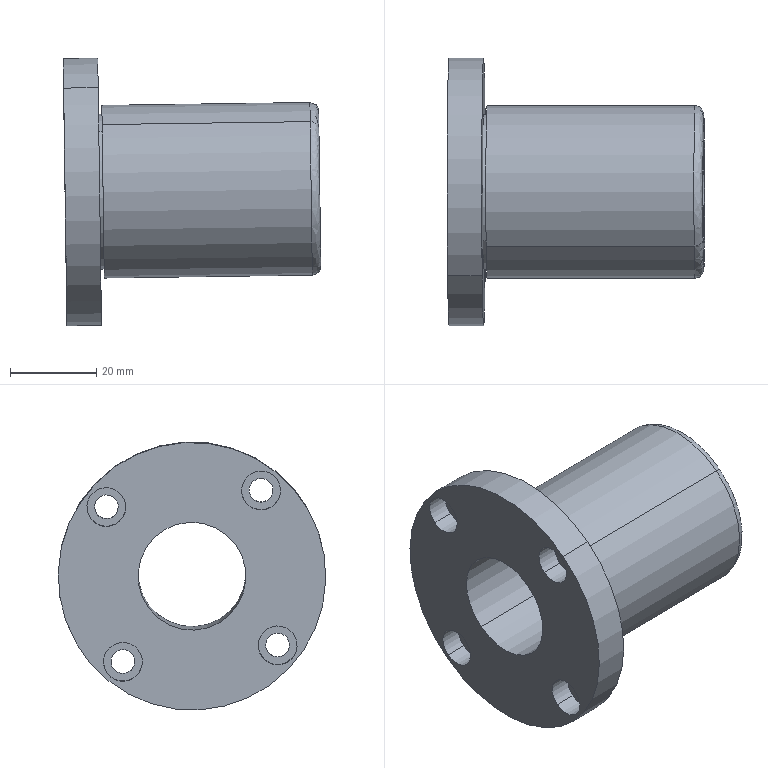Component | SolidWorks | DA-0220-LHFR25-18 | 1 solid | 34 faces | box 59.68 x 62 x 62.11 mm | volume 57411 mm3 | cylinder 24 | plane 8 | spline 2 | commonest cylinder face diameters 5.5 x8 9 x8 40 x2 36 x2 25 x2 62 x2
STEP:
#1=CARTESIAN_POINT('',(34.201,-7.018,18.749));
#2=VERTEX_POINT('',#1);
#3=CARTESIAN_POINT('',(34.218,-6.029,17.524));
#4=VERTEX_POINT('',#3);
#5=CARTESIAN_POINT('',(34.209,-6.524,18.137));
#6=DIRECTION('',(-0.9999,-0.000404,-0.01395));
#7=DIRECTION('',(-0.01061,-0.628,0.7781));
#8=AXIS2_PLACEMENT_3D('',#5,#6,#7);
#9=CIRCLE('',#8,0.7874);
#10=EDGE_CURVE('',#2,#4,#9,.T.);
#11=ORIENTED_EDGE('',*,*,#10,.F.);
#12=CARTESIAN_POINT('',(34.28,-6.969,18.689));
#13=VERTEX_POINT('',#12);
#14=CARTESIAN_POINT('',(34.202,-6.969,18.688));
#15=DIRECTION('',(-0.009077,0.7782,0.6279));
#16=DIRECTION('',(-0.01061,-0.628,0.7781));
#17=AXIS2_PLACEMENT_3D('',#14,#15,#16);
#18=CIRCLE('',#17,0.07874);
#19=EDGE_CURVE('',#2,#13,#18,.T.);
#20=ORIENTED_EDGE('',*,*,#19,.T.);
#21=CARTESIAN_POINT('',(34.295,-6.079,17.586));
#22=VERTEX_POINT('',#21);
#23=CARTESIAN_POINT('',(34.28,-6.969,18.689));
#24=CARTESIAN_POINT('',(34.268,-5.866,19.579));
#25=CARTESIAN_POINT('',(34.283,-4.976,18.476));
#26=CARTESIAN_POINT('',(34.295,-6.079,17.586));
#27=(BOUNDED_CURVE()B_SPLINE_CURVE(3,(#23,#24,#25,#26),.UNSPECIFIED.,.F.,.F.)B_SPLINE_CURVE_WITH_KNOTS((4,4),(0.,1.),.UNSPECIFIED.)CURVE()GEOMETRIC_REPRESENTATION_ITEM()RATIONAL_B_SPLINE_CURVE((1.,0.3333,0.3333,1.))REPRESENTATION_ITEM(''));
#28=EDGE_CURVE('',#13,#22,#27,.T.);
#29=ORIENTED_EDGE('',*,*,#28,.T.);
#30=CARTESIAN_POINT('',(34.217,-6.079,17.585));
#31=DIRECTION('',(0.009077,-0.7782,-0.6279));
#32=DIRECTION('',(0.01061,0.628,-0.7781));
#33=AXIS2_PLACEMENT_3D('',#30,#31,#32);
#34=CIRCLE('',#33,0.07874);
#35=EDGE_CURVE('',#4,#22,#34,.T.);
#36=ORIENTED_EDGE('',*,*,#35,.F.);
#37=EDGE_LOOP('',(#11,#20,#29,#36));
#38=FACE_OUTER_BOUND('',#37,.T.);
#39=CARTESIAN_POINT('',(34.201,-7.018,18.749));
#40=CARTESIAN_POINT('',(34.187,-5.793,19.738));
#41=CARTESIAN_POINT('',(34.203,-4.804,18.513));
#42=CARTESIAN_POINT('',(34.218,-6.029,17.524));
#43=CARTESIAN_POINT('',(34.247,-7.018,18.75));
#44=CARTESIAN_POINT('',(34.233,-5.793,19.739));
#45=CARTESIAN_POINT('',(34.249,-4.804,18.513));
#46=CARTESIAN_POINT('',(34.264,-6.029,17.525));
#47=CARTESIAN_POINT('',(34.28,-6.998,18.725));
#48=CARTESIAN_POINT('',(34.266,-5.823,19.673));
#49=CARTESIAN_POINT('',(34.282,-4.875,18.498));
#50=CARTESIAN_POINT('',(34.296,-6.05,17.55));
#51=CARTESIAN_POINT('',(34.28,-6.969,18.689));
#52=CARTESIAN_POINT('',(34.268,-5.866,19.579));
#53=CARTESIAN_POINT('',(34.283,-4.976,18.476));
#54=CARTESIAN_POINT('',(34.295,-6.079,17.586));
#55=(BOUNDED_SURFACE()B_SPLINE_SURFACE(3,3,((#39,#40,#41,#42),(#43,#44,#45,#46),(#47,#48,#49,#50),(#51,#52,#53,#54)),.UNSPECIFIED.,.F.,.F.,.T.)B_SPLINE_SURFACE_WITH_KNOTS((4,4),(4,4),(0.,1.),(0.,1.),.UNSPECIFIED.)GEOMETRIC_REPRESENTATION_ITEM()RATIONAL_B_SPLINE_SURFACE(((1.,0.3333,0.3333,1.),(0.8047,0.2682,0.2682,0.8047),(0.8047,0.2682,0.2682,0.8047),(1.,0.3333,0.3333,1.)))REPRESENTATION_ITEM('')SURFACE());
#56=ADVANCED_FACE('',(#38),#55,.T.);
#57=CARTESIAN_POINT('',(32.303,-7.019,18.723));
#58=VERTEX_POINT('',#57);
#59=CARTESIAN_POINT('',(32.32,-6.03,17.497));
#60=VERTEX_POINT('',#59);
#61=CARTESIAN_POINT('',(32.312,-6.524,18.11));
#62=DIRECTION('',(0.9999,0.000404,0.01395));
#63=DIRECTION('',(-0.01061,-0.628,0.7781));
#64=AXIS2_PLACEMENT_3D('',#61,#62,#63);
#65=CIRCLE('',#64,0.7874);
#66=EDGE_CURVE('',#58,#60,#65,.T.);
#67=ORIENTED_EDGE('',*,*,#66,.T.);
#68=CARTESIAN_POINT('',(33.269,-6.03,17.511));
#69=DIRECTION('',(0.9999,0.000404,0.01395));
#70=VECTOR('',#69,39.37);
#71=LINE('',#68,#70);
#72=EDGE_CURVE('',#60,#4,#71,.T.);
#73=ORIENTED_EDGE('',*,*,#72,.T.);
#74=CARTESIAN_POINT('',(34.209,-6.524,18.137));
#75=DIRECTION('',(-0.9999,-0.000404,-0.01395));
#76=DIRECTION('',(-0.01061,-0.628,0.7781));
#77=AXIS2_PLACEMENT_3D('',#74,#75,#76);
#78=CIRCLE('',#77,0.7874);
#79=EDGE_CURVE('',#4,#2,#78,.T.);
#80=ORIENTED_EDGE('',*,*,#79,.T.);
#81=CARTESIAN_POINT('',(33.252,-7.018,18.736));
#82=DIRECTION('',(0.9999,0.000404,0.01395));
#83=VECTOR('',#82,39.37);
#84=LINE('',#81,#83);
#85=EDGE_CURVE('',#58,#2,#84,.T.);
#86=ORIENTED_EDGE('',*,*,#85,.F.);
#87=EDGE_LOOP('',(#67,#73,#80,#86));
#88=FACE_OUTER_BOUND('',#87,.T.);
#89=CARTESIAN_POINT('',(33.26,-6.524,18.123));
#90=DIRECTION('',(0.9999,0.000404,0.01395));
#91=DIRECTION('',(-0.01061,-0.628,0.7781));
#92=AXIS2_PLACEMENT_3D('',#89,#90,#91);
#93=CYLINDRICAL_SURFACE('',#92,0.7874);
#94=ADVANCED_FACE('',(#88),#93,.T.);
#95=CARTESIAN_POINT('',(32.273,-6.969,18.661));
#96=VERTEX_POINT('',#95);
#97=CARTESIAN_POINT('',(32.288,-6.079,17.558));
#98=VERTEX_POINT('',#97);
#99=CARTESIAN_POINT('',(32.28,-6.524,18.11));
#100=DIRECTION('',(0.9999,0.000404,0.01395));
#101=DIRECTION('',(-0.01061,-0.628,0.7781));
#102=AXIS2_PLACEMENT_3D('',#99,#100,#101);
#103=CIRCLE('',#102,0.7087);
#104=EDGE_CURVE('',#96,#98,#103,.T.);
#105=ORIENTED_EDGE('',*,*,#104,.T.);
#106=CARTESIAN_POINT('',(32.319,-6.079,17.559));
#107=VERTEX_POINT('',#106);
#108=CARTESIAN_POINT('',(32.304,-6.079,17.558));
#109=DIRECTION('',(0.9999,0.000404,0.01395));
#110=VECTOR('',#109,39.37);
#111=LINE('',#108,#110);
#112=EDGE_CURVE('',#98,#107,#111,.T.);
#113=ORIENTED_EDGE('',*,*,#112,.T.);
#114=CARTESIAN_POINT('',(32.304,-6.969,18.662));
#115=VERTEX_POINT('',#114);
#116=CARTESIAN_POINT('',(32.312,-6.524,18.11));
#117=DIRECTION('',(0.9999,0.000404,0.01395));
#118=DIRECTION('',(-0.01061,-0.628,0.7781));
#119=AXIS2_PLACEMENT_3D('',#116,#117,#118);
#120=CIRCLE('',#119,0.7087);
#121=EDGE_CURVE('',#115,#107,#120,.T.);
#122=ORIENTED_EDGE('',*,*,#121,.F.);
#123=CARTESIAN_POINT('',(32.289,-6.969,18.661));
#124=DIRECTION('',(0.9999,0.000404,0.01395));
#125=VECTOR('',#124,39.37);
#126=LINE('',#123,#125);
#127=EDGE_CURVE('',#96,#115,#126,.T.);
#128=ORIENTED_EDGE('',*,*,#127,.F.);
#129=EDGE_LOOP('',(#105,#113,#122,#128));
#130=FACE_OUTER_BOUND('',#129,.T.);
#131=CARTESIAN_POINT('',(32.296,-6.524,18.11));
#132=DIRECTION('',(0.9999,0.000404,0.01395));
#133=DIRECTION('',(-0.01061,-0.628,0.7781));
#134=AXIS2_PLACEMENT_3D('',#131,#132,#133);
#135=CYLINDRICAL_SURFACE('',#134,0.7087);
#136=ADVANCED_FACE('',(#130),#135,.T.);
#137=CARTESIAN_POINT('',(31.971,-6.215,17.722));
#138=VERTEX_POINT('',#137);
#139=CARTESIAN_POINT('',(31.96,-6.834,18.488));
#140=VERTEX_POINT('',#139);
#141=CARTESIAN_POINT('',(31.965,-6.525,18.105));
#142=DIRECTION('',(0.9999,0.000404,0.01395));
#143=DIRECTION('',(-0.01061,-0.628,0.7781));
#144=AXIS2_PLACEMENT_3D('',#141,#142,#143);
#145=CIRCLE('',#144,0.4921);
#146=EDGE_CURVE('',#138,#140,#145,.T.);
#147=ORIENTED_EDGE('',*,*,#146,.F.);
#148=CARTESIAN_POINT('',(34.293,-6.215,17.755));
#149=VERTEX_POINT('',#148);
#150=CARTESIAN_POINT('',(33.132,-6.215,17.739));
#151=DIRECTION('',(0.9999,0.000404,0.01395));
#152=VECTOR('',#151,39.37);
#153=LINE('',#150,#152);
#154=EDGE_CURVE('',#138,#149,#153,.T.);
#155=ORIENTED_EDGE('',*,*,#154,.T.);
#156=CARTESIAN_POINT('',(34.283,-6.833,18.521));
#157=VERTEX_POINT('',#156);
#158=CARTESIAN_POINT('',(34.288,-6.524,18.138));
#159=DIRECTION('',(-0.9999,-0.000404,-0.01395));
#160=DIRECTION('',(-0.01061,-0.628,0.7781));
#161=AXIS2_PLACEMENT_3D('',#158,#159,#160);
#162=CIRCLE('',#161,0.4921);
#163=EDGE_CURVE('',#157,#149,#162,.T.);
#164=ORIENTED_EDGE('',*,*,#163,.F.);
#165=CARTESIAN_POINT('',(33.121,-6.833,18.504));
#166=DIRECTION('',(0.9999,0.000404,0.01395));
#167=VECTOR('',#166,39.37);
#168=LINE('',#165,#167);
#169=EDGE_CURVE('',#140,#157,#168,.T.);
#170=ORIENTED_EDGE('',*,*,#169,.F.);
#171=EDGE_LOOP('',(#147,#155,#164,#170));
#172=FACE_OUTER_BOUND('',#171,.T.);
#173=CARTESIAN_POINT('',(33.127,-6.524,18.122));
#174=DIRECTION('',(0.9999,0.000404,0.01395));
#175=DIRECTION('',(-0.01061,-0.628,0.7781));
#176=AXIS2_PLACEMENT_3D('',#173,#174,#175);
#177=CYLINDRICAL_SURFACE('',#176,0.4921);
#178=ADVANCED_FACE('',(#172),#177,.F.);
#179=CARTESIAN_POINT('',(31.978,-5.758,17.156));
#180=VERTEX_POINT('',#179);
#181=CARTESIAN_POINT('',(31.952,-7.291,19.055));
#182=VERTEX_POINT('',#181);
#183=CARTESIAN_POINT('',(31.965,-6.525,18.105));
#184=DIRECTION('',(-0.9999,-0.000404,-0.01395));
#185=DIRECTION('',(-0.01061,-0.628,0.7781));
#186=AXIS2_PLACEMENT_3D('',#183,#184,#185);
#187=CIRCLE('',#186,1.22);
#188=EDGE_CURVE('',#180,#182,#187,.T.);
#189=ORIENTED_EDGE('',*,*,#188,.F.);
#190=CARTESIAN_POINT('',(32.293,-5.758,17.16));
#191=VERTEX_POINT('',#190);
#192=CARTESIAN_POINT('',(32.136,-5.758,17.158));
#193=DIRECTION('',(0.9999,0.000404,0.01395));
#194=VECTOR('',#193,39.37);
#195=LINE('',#192,#194);
#196=EDGE_CURVE('',#180,#191,#195,.T.);
#197=ORIENTED_EDGE('',*,*,#196,.T.);
#198=CARTESIAN_POINT('',(32.267,-7.291,19.059));
#199=VERTEX_POINT('',#198);
#200=CARTESIAN_POINT('',(32.28,-6.524,18.11));
#201=DIRECTION('',(0.9999,0.000404,0.01395));
#202=DIRECTION('',(-0.01061,-0.628,0.7781));
#203=AXIS2_PLACEMENT_3D('',#200,#201,#202);
#204=CIRCLE('',#203,1.22);
#205=EDGE_CURVE('',#199,#191,#204,.T.);
#206=ORIENTED_EDGE('',*,*,#205,.F.);
#207=CARTESIAN_POINT('',(32.11,-7.291,19.057));
#208=DIRECTION('',(0.9999,0.000404,0.01395));
#209=VECTOR('',#208,39.37);
#210=LINE('',#207,#209);
#211=EDGE_CURVE('',#182,#199,#210,.T.);
#212=ORIENTED_EDGE('',*,*,#211,.F.);
#213=EDGE_LOOP('',(#189,#197,#206,#212));
#214=FACE_OUTER_BOUND('',#213,.T.);
#215=CARTESIAN_POINT('',(32.123,-6.524,18.107));
#216=DIRECTION('',(0.9999,0.000404,0.01395));
#217=DIRECTION('',(-0.01061,-0.628,0.7781));
#218=AXIS2_PLACEMENT_3D('',#215,#216,#217);
#219=CYLINDRICAL_SURFACE('',#218,1.22);
#220=ADVANCED_FACE('',(#214),#219,.T.);
#221=CARTESIAN_POINT('',(32.176,-7.238,17.393));
#222=VERTEX_POINT('',#221);
#223=CARTESIAN_POINT('',(32.174,-7.374,17.562));
#224=VERTEX_POINT('',#223);
#225=CARTESIAN_POINT('',(32.175,-7.306,17.478));
#226=DIRECTION('',(0.9999,0.000404,0.01395));
#227=DIRECTION('',(-0.01061,-0.628,0.7781));
#228=AXIS2_PLACEMENT_3D('',#225,#226,#227);
#229=CIRCLE('',#228,0.1083);
#230=EDGE_CURVE('',#222,#224,#229,.T.);
#231=ORIENTED_EDGE('',*,*,#230,.F.);
#232=CARTESIAN_POINT('',(32.291,-7.238,17.395));
#233=VERTEX_POINT('',#232);
#234=CARTESIAN_POINT('',(32.233,-7.238,17.394));
#235=DIRECTION('',(0.9999,0.000404,0.01395));
#236=VECTOR('',#235,39.37);
#237=LINE('',#234,#236);
#238=EDGE_CURVE('',#222,#233,#237,.T.);
#239=ORIENTED_EDGE('',*,*,#238,.T.);
#240=CARTESIAN_POINT('',(32.288,-7.374,17.564));
#241=VERTEX_POINT('',#240);
#242=CARTESIAN_POINT('',(32.289,-7.306,17.479));
#243=DIRECTION('',(-0.9999,-0.000404,-0.01395));
#244=DIRECTION('',(-0.01061,-0.628,0.7781));
#245=AXIS2_PLACEMENT_3D('',#242,#243,#244);
#246=CIRCLE('',#245,0.1083);
#247=EDGE_CURVE('',#241,#233,#246,.T.);
#248=ORIENTED_EDGE('',*,*,#247,.F.);
#249=CARTESIAN_POINT('',(32.231,-7.374,17.563));
#250=DIRECTION('',(0.9999,0.000404,0.01395));
#251=VECTOR('',#250,39.37);
#252=LINE('',#249,#251);
#253=EDGE_CURVE('',#224,#241,#252,.T.);
#254=ORIENTED_EDGE('',*,*,#253,.F.);
#255=EDGE_LOOP('',(#231,#239,#248,#254));
#256=FACE_OUTER_BOUND('',#255,.T.);
#257=CARTESIAN_POINT('',(32.232,-7.306,17.478));
#258=DIRECTION('',(0.9999,0.000404,0.01395));
#259=DIRECTION('',(-0.01061,-0.628,0.7781));
#260=AXIS2_PLACEMENT_3D('',#257,#258,#259);
#261=CYLINDRICAL_SURFACE('',#260,0.1083);
#262=ADVANCED_FACE('',(#256),#261,.F.);
#263=CARTESIAN_POINT('',(32.157,-7.087,18.805));
#264=VERTEX_POINT('',#263);
#265=CARTESIAN_POINT('',(32.154,-7.223,18.974));
#266=VERTEX_POINT('',#265);
#267=CARTESIAN_POINT('',(32.155,-7.155,18.889));
#268=DIRECTION('',(0.9999,0.000404,0.01395));
#269=DIRECTION('',(-0.01061,-0.628,0.7781));
#270=AXIS2_PLACEMENT_3D('',#267,#268,#269);
#271=CIRCLE('',#270,0.1083);
#272=EDGE_CURVE('',#264,#266,#271,.T.);
#273=ORIENTED_EDGE('',*,*,#272,.F.);
#274=CARTESIAN_POINT('',(32.271,-7.087,18.807));
#275=VERTEX_POINT('',#274);
#276=CARTESIAN_POINT('',(32.214,-7.087,18.806));
#277=DIRECTION('',(0.9999,0.000404,0.01395));
#278=VECTOR('',#277,39.37);
#279=LINE('',#276,#278);
#280=EDGE_CURVE('',#264,#275,#279,.T.);
#281=ORIENTED_EDGE('',*,*,#280,.T.);
#282=CARTESIAN_POINT('',(32.268,-7.223,18.975));
#283=VERTEX_POINT('',#282);
#284=CARTESIAN_POINT('',(32.27,-7.155,18.891));
#285=DIRECTION('',(-0.9999,-0.000404,-0.01395));
#286=DIRECTION('',(-0.01061,-0.628,0.7781));
#287=AXIS2_PLACEMENT_3D('',#284,#285,#286);
#288=CIRCLE('',#287,0.1083);
#289=EDGE_CURVE('',#283,#275,#288,.T.);
#290=ORIENTED_EDGE('',*,*,#289,.F.);
#291=CARTESIAN_POINT('',(32.211,-7.223,18.974));
#292=DIRECTION('',(0.9999,0.000404,0.01395));
#293=VECTOR('',#292,39.37);
#294=LINE('',#291,#293);
#295=EDGE_CURVE('',#266,#283,#294,.T.);
#296=ORIENTED_EDGE('',*,*,#295,.F.);
#297=EDGE_LOOP('',(#273,#281,#290,#296));
#298=FACE_OUTER_BOUND('',#297,.T.);
#299=CARTESIAN_POINT('',(32.213,-7.155,18.89));
#300=DIRECTION('',(0.9999,0.000404,0.01395));
#301=DIRECTION('',(-0.01061,-0.628,0.7781));
#302=AXIS2_PLACEMENT_3D('',#299,#300,#301);
#303=CYLINDRICAL_SURFACE('',#302,0.1083);
#304=ADVANCED_FACE('',(#298),#303,.F.);
#305=CARTESIAN_POINT('',(32.158,-5.675,18.654));
#306=VERTEX_POINT('',#305);
#307=CARTESIAN_POINT('',(32.156,-5.811,18.823));
#308=VERTEX_POINT('',#307);
#309=CARTESIAN_POINT('',(32.157,-5.743,18.738));
#310=DIRECTION('',(0.9999,0.000404,0.01395));
#311=DIRECTION('',(-0.01061,-0.628,0.7781));
#312=AXIS2_PLACEMENT_3D('',#309,#310,#311);
#313=CIRCLE('',#312,0.1083);
#314=EDGE_CURVE('',#306,#308,#313,.T.);
#315=ORIENTED_EDGE('',*,*,#314,.F.);
#316=CARTESIAN_POINT('',(32.272,-5.675,18.656));
#317=VERTEX_POINT('',#316);
#318=CARTESIAN_POINT('',(32.215,-5.675,18.655));
#319=DIRECTION('',(0.9999,0.000404,0.01395));
#320=VECTOR('',#319,39.37);
#321=LINE('',#318,#320);
#322=EDGE_CURVE('',#306,#317,#321,.T.);
#323=ORIENTED_EDGE('',*,*,#322,.T.);
#324=CARTESIAN_POINT('',(32.27,-5.811,18.824));
#325=VERTEX_POINT('',#324);
#326=CARTESIAN_POINT('',(32.271,-5.743,18.74));
#327=DIRECTION('',(-0.9999,-0.000404,-0.01395));
#328=DIRECTION('',(-0.01061,-0.628,0.7781));
#329=AXIS2_PLACEMENT_3D('',#326,#327,#328);
#330=CIRCLE('',#329,0.1083);
#331=EDGE_CURVE('',#325,#317,#330,.T.);
#332=ORIENTED_EDGE('',*,*,#331,.F.);
#333=CARTESIAN_POINT('',(32.213,-5.811,18.824));
#334=DIRECTION('',(0.9999,0.000404,0.01395));
#335=VECTOR('',#334,39.37);
#336=LINE('',#333,#335);
#337=EDGE_CURVE('',#308,#325,#336,.T.);
#338=ORIENTED_EDGE('',*,*,#337,.F.);
#339=EDGE_LOOP('',(#315,#323,#332,#338));
#340=FACE_OUTER_BOUND('',#339,.T.);
#341=CARTESIAN_POINT('',(32.214,-5.743,18.739));
#342=DIRECTION('',(0.9999,0.000404,0.01395));
#343=DIRECTION('',(-0.01061,-0.628,0.7781));
#344=AXIS2_PLACEMENT_3D('',#341,#342,#343);
#345=CYLINDRICAL_SURFACE('',#344,0.1083);
#346=ADVANCED_FACE('',(#340),#345,.F.);
#347=CARTESIAN_POINT('',(32.178,-5.826,17.243));
#348=VERTEX_POINT('',#347);
#349=CARTESIAN_POINT('',(32.176,-5.962,17.411));
#350=VERTEX_POINT('',#349);
#351=CARTESIAN_POINT('',(32.177,-5.894,17.327));
#352=DIRECTION('',(0.9999,0.000404,0.01395));
#353=DIRECTION('',(-0.01061,-0.628,0.7781));
#354=AXIS2_PLACEMENT_3D('',#351,#352,#353);
#355=CIRCLE('',#354,0.1083);
#356=EDGE_CURVE('',#348,#350,#355,.T.);
#357=ORIENTED_EDGE('',*,*,#356,.F.);
#358=CARTESIAN_POINT('',(32.292,-5.826,17.244));
#359=VERTEX_POINT('',#358);
#360=CARTESIAN_POINT('',(32.235,-5.826,17.243));
#361=DIRECTION('',(0.9999,0.000404,0.01395));
#362=VECTOR('',#361,39.37);
#363=LINE('',#360,#362);
#364=EDGE_CURVE('',#348,#359,#363,.T.);
#365=ORIENTED_EDGE('',*,*,#364,.T.);
#366=CARTESIAN_POINT('',(32.29,-5.962,17.413));
#367=VERTEX_POINT('',#366);
#368=CARTESIAN_POINT('',(32.291,-5.894,17.328));
#369=DIRECTION('',(-0.9999,-0.000404,-0.01395));
#370=DIRECTION('',(-0.01061,-0.628,0.7781));
#371=AXIS2_PLACEMENT_3D('',#368,#369,#370);
#372=CIRCLE('',#371,0.1083);
#373=EDGE_CURVE('',#367,#359,#372,.T.);
#374=ORIENTED_EDGE('',*,*,#373,.F.);
#375=CARTESIAN_POINT('',(32.233,-5.962,17.412));
#376=DIRECTION('',(0.9999,0.000404,0.01395));
#377=VECTOR('',#376,39.37);
#378=LINE('',#375,#377);
#379=EDGE_CURVE('',#350,#367,#378,.T.);
#380=ORIENTED_EDGE('',*,*,#379,.F.);
#381=EDGE_LOOP('',(#357,#365,#374,#380));
#382=FACE_OUTER_BOUND('',#381,.T.);
#383=CARTESIAN_POINT('',(32.234,-5.894,17.328));
#384=DIRECTION('',(0.9999,0.000404,0.01395));
#385=DIRECTION('',(-0.01061,-0.628,0.7781));
#386=AXIS2_PLACEMENT_3D('',#383,#384,#385);
#387=CYLINDRICAL_SURFACE('',#386,0.1083);
#388=ADVANCED_FACE('',(#382),#387,.F.);
#389=CARTESIAN_POINT('',(31.976,-7.195,17.337));
#390=VERTEX_POINT('',#389);
#391=CARTESIAN_POINT('',(31.973,-7.417,17.613));
#392=VERTEX_POINT('',#391);
#393=CARTESIAN_POINT('',(31.974,-7.306,17.475));
#394=DIRECTION('',(0.9999,0.000404,0.01395));
#395=DIRECTION('',(-0.01061,-0.628,0.7781));
#396=AXIS2_PLACEMENT_3D('',#393,#394,#395);
#397=CIRCLE('',#396,0.1772);
#398=EDGE_CURVE('',#390,#392,#397,.T.);
#399=ORIENTED_EDGE('',*,*,#398,.F.);
#400=CARTESIAN_POINT('',(32.177,-7.194,17.34));
#401=VERTEX_POINT('',#400);
#402=CARTESIAN_POINT('',(32.077,-7.195,17.338));
#403=DIRECTION('',(0.9999,0.000404,0.01395));
#404=VECTOR('',#403,39.37);
#405=LINE('',#402,#404);
#406=EDGE_CURVE('',#390,#401,#405,.T.);
#407=ORIENTED_EDGE('',*,*,#406,.T.);
#408=CARTESIAN_POINT('',(32.173,-7.417,17.616));
#409=VERTEX_POINT('',#408);
#410=CARTESIAN_POINT('',(32.175,-7.306,17.478));
#411=DIRECTION('',(-0.9999,-0.000404,-0.01395));
#412=DIRECTION('',(-0.01061,-0.628,0.7781));
#413=AXIS2_PLACEMENT_3D('',#410,#411,#412);
#414=CIRCLE('',#413,0.1772);
#415=EDGE_CURVE('',#409,#401,#414,.T.);
#416=ORIENTED_EDGE('',*,*,#415,.F.);
#417=CARTESIAN_POINT('',(32.073,-7.417,17.614));
#418=DIRECTION('',(0.9999,0.000404,0.01395));
#419=VECTOR('',#418,39.37);
#420=LINE('',#417,#419);
#421=EDGE_CURVE('',#392,#409,#420,.T.);
#422=ORIENTED_EDGE('',*,*,#421,.F.);
#423=EDGE_LOOP('',(#399,#407,#416,#422));
#424=FACE_OUTER_BOUND('',#423,.T.);
#425=CARTESIAN_POINT('',(32.075,-7.306,17.476));
#426=DIRECTION('',(0.9999,0.000404,0.01395));
#427=DIRECTION('',(-0.01061,-0.628,0.7781));
#428=AXIS2_PLACEMENT_3D('',#425,#426,#427);
#429=CYLINDRICAL_SURFACE('',#428,0.1772);
#430=ADVANCED_FACE('',(#424),#429,.F.);
#431=CARTESIAN_POINT('',(31.957,-7.044,18.749));
#432=VERTEX_POINT('',#431);
#433=CARTESIAN_POINT('',(31.953,-7.266,19.024));
#434=VERTEX_POINT('',#433);
#435=CARTESIAN_POINT('',(31.955,-7.155,18.887));
#436=DIRECTION('',(0.9999,0.000404,0.01395));
#437=DIRECTION('',(-0.01061,-0.628,0.7781));
#438=AXIS2_PLACEMENT_3D('',#435,#436,#437);
#439=CIRCLE('',#438,0.1772);
#440=EDGE_CURVE('',#432,#434,#439,.T.);
#441=ORIENTED_EDGE('',*,*,#440,.F.);
#442=CARTESIAN_POINT('',(32.157,-7.044,18.751));
#443=VERTEX_POINT('',#442);
#444=CARTESIAN_POINT('',(32.057,-7.044,18.75));
#445=DIRECTION('',(0.9999,0.000404,0.01395));
#446=VECTOR('',#445,39.37);
#447=LINE('',#444,#446);
#448=EDGE_CURVE('',#432,#443,#447,.T.);
#449=ORIENTED_EDGE('',*,*,#448,.T.);
#450=CARTESIAN_POINT('',(32.154,-7.266,19.027));
#451=VERTEX_POINT('',#450);
#452=CARTESIAN_POINT('',(32.155,-7.155,18.889));
#453=DIRECTION('',(-0.9999,-0.000404,-0.01395));
#454=DIRECTION('',(-0.01061,-0.628,0.7781));
#455=AXIS2_PLACEMENT_3D('',#452,#453,#454);
#456=CIRCLE('',#455,0.1772);
#457=EDGE_CURVE('',#451,#443,#456,.T.);
#458=ORIENTED_EDGE('',*,*,#457,.F.);
#459=CARTESIAN_POINT('',(32.053,-7.266,19.026));
#460=DIRECTION('',(0.9999,0.000404,0.01395));
#461=VECTOR('',#460,39.37);
#462=LINE('',#459,#461);
#463=EDGE_CURVE('',#434,#451,#462,.T.);
#464=ORIENTED_EDGE('',*,*,#463,.F.);
#465=EDGE_LOOP('',(#441,#449,#458,#464));
#466=FACE_OUTER_BOUND('',#465,.T.);
#467=CARTESIAN_POINT('',(32.055,-7.155,18.888));
#468=DIRECTION('',(0.9999,0.000404,0.01395));
#469=DIRECTION('',(-0.01061,-0.628,0.7781));
#470=AXIS2_PLACEMENT_3D('',#467,#468,#469);
#471=CYLINDRICAL_SURFACE('',#470,0.1772);
#472=ADVANCED_FACE('',(#466),#471,.F.);
#473=CARTESIAN_POINT('',(31.958,-5.632,18.598));
#474=VERTEX_POINT('',#473);
#475=CARTESIAN_POINT('',(31.954,-5.855,18.874));
#476=VERTEX_POINT('',#475);
#477=CARTESIAN_POINT('',(31.956,-5.743,18.736));
#478=DIRECTION('',(0.9999,0.000404,0.01395));
#479=DIRECTION('',(-0.01061,-0.628,0.7781));
#480=AXIS2_PLACEMENT_3D('',#477,#478,#479);
#481=CIRCLE('',#480,0.1772);
#482=EDGE_CURVE('',#474,#476,#481,.T.);
#483=ORIENTED_EDGE('',*,*,#482,.F.);
#484=CARTESIAN_POINT('',(32.159,-5.632,18.601));
#485=VERTEX_POINT('',#484);
#486=CARTESIAN_POINT('',(32.058,-5.632,18.599));
#487=DIRECTION('',(0.9999,0.000404,0.01395));
#488=VECTOR('',#487,39.37);
#489=LINE('',#486,#488);
#490=EDGE_CURVE('',#474,#485,#489,.T.);
#491=ORIENTED_EDGE('',*,*,#490,.T.);
#492=CARTESIAN_POINT('',(32.155,-5.854,18.876));
#493=VERTEX_POINT('',#492);
#494=CARTESIAN_POINT('',(32.157,-5.743,18.738));
#495=DIRECTION('',(-0.9999,-0.000404,-0.01395));
#496=DIRECTION('',(-0.01061,-0.628,0.7781));
#497=AXIS2_PLACEMENT_3D('',#494,#495,#496);
#498=CIRCLE('',#497,0.1772);
#499=EDGE_CURVE('',#493,#485,#498,.T.);
#500=ORIENTED_EDGE('',*,*,#499,.F.);
#501=CARTESIAN_POINT('',(32.055,-5.854,18.875));
#502=DIRECTION('',(0.9999,0.000404,0.01395));
#503=VECTOR('',#502,39.37);
#504=LINE('',#501,#503);
#505=EDGE_CURVE('',#476,#493,#504,.T.);
#506=ORIENTED_EDGE('',*,*,#505,.F.);
#507=EDGE_LOOP('',(#483,#491,#500,#506));
#508=FACE_OUTER_BOUND('',#507,.T.);
#509=CARTESIAN_POINT('',(32.057,-5.743,18.737));
#510=DIRECTION('',(0.9999,0.000404,0.01395));
#511=DIRECTION('',(-0.01061,-0.628,0.7781));
#512=AXIS2_PLACEMENT_3D('',#509,#510,#511);
#513=CYLINDRICAL_SURFACE('',#512,0.1772);
#514=ADVANCED_FACE('',(#508),#513,.F.);
#515=CARTESIAN_POINT('',(31.978,-5.783,17.186));
#516=VERTEX_POINT('',#515);
#517=CARTESIAN_POINT('',(31.974,-6.005,17.462));
#518=VERTEX_POINT('',#517);
#519=CARTESIAN_POINT('',(31.976,-5.894,17.324));
#520=DIRECTION('',(0.9999,0.000404,0.01395));
#521=DIRECTION('',(-0.01061,-0.628,0.7781));
#522=AXIS2_PLACEMENT_3D('',#519,#520,#521);
#523=CIRCLE('',#522,0.1772);
#524=EDGE_CURVE('',#516,#518,#523,.T.);
#525=ORIENTED_EDGE('',*,*,#524,.F.);
#526=CARTESIAN_POINT('',(32.179,-5.783,17.189));
#527=VERTEX_POINT('',#526);
#528=CARTESIAN_POINT('',(32.078,-5.783,17.188));
#529=DIRECTION('',(0.9999,0.000404,0.01395));
#530=VECTOR('',#529,39.37);
#531=LINE('',#528,#530);
#532=EDGE_CURVE('',#516,#527,#531,.T.);
#533=ORIENTED_EDGE('',*,*,#532,.T.);
#534=CARTESIAN_POINT('',(32.175,-6.005,17.465));
#535=VERTEX_POINT('',#534);
#536=CARTESIAN_POINT('',(32.177,-5.894,17.327));
#537=DIRECTION('',(-0.9999,-0.000404,-0.01395));
#538=DIRECTION('',(-0.01061,-0.628,0.7781));
#539=AXIS2_PLACEMENT_3D('',#536,#537,#538);
#540=CIRCLE('',#539,0.1772);
#541=EDGE_CURVE('',#535,#527,#540,.T.);
#542=ORIENTED_EDGE('',*,*,#541,.F.);
#543=CARTESIAN_POINT('',(32.075,-6.005,17.463));
#544=DIRECTION('',(0.9999,0.000404,0.01395));
#545=VECTOR('',#544,39.37);
#546=LINE('',#543,#545);
#547=EDGE_CURVE('',#518,#535,#546,.T.);
#548=ORIENTED_EDGE('',*,*,#547,.F.);
#549=EDGE_LOOP('',(#525,#533,#542,#548));
#550=FACE_OUTER_BOUND('',#549,.T.);
#551=CARTESIAN_POINT('',(32.076,-5.894,17.325));
#552=DIRECTION('',(0.9999,0.000404,0.01395));
#553=DIRECTION('',(-0.01061,-0.628,0.7781));
#554=AXIS2_PLACEMENT_3D('',#551,#552,#553);
#555=CYLINDRICAL_SURFACE('',#554,0.1772);
#556=ADVANCED_FACE('',(#550),#555,.F.);
#557=ORIENTED_EDGE('',*,*,#72,.F.);
#558=CARTESIAN_POINT('',(32.312,-6.524,18.11));
#559=DIRECTION('',(0.9999,0.000404,0.01395));
#560=DIRECTION('',(-0.01061,-0.628,0.7781));
#561=AXIS2_PLACEMENT_3D('',#558,#559,#560);
#562=CIRCLE('',#561,0.7874);
#563=EDGE_CURVE('',#60,#58,#562,.T.);
#564=ORIENTED_EDGE('',*,*,#563,.T.);
#565=ORIENTED_EDGE('',*,*,#85,.T.);
#566=ORIENTED_EDGE('',*,*,#10,.T.);
#567=EDGE_LOOP('',(#557,#564,#565,#566));
#568=FACE_OUTER_BOUND('',#567,.T.);
#569=CARTESIAN_POINT('',(33.26,-6.524,18.123));
#570=DIRECTION('',(0.9999,0.000404,0.01395));
#571=DIRECTION('',(-0.01061,-0.628,0.7781));
#572=AXIS2_PLACEMENT_3D('',#569,#570,#571);
#573=CYLINDRICAL_SURFACE('',#572,0.7874);
#574=ADVANCED_FACE('',(#568),#573,.T.);
#575=ORIENTED_EDGE('',*,*,#19,.F.);
#576=ORIENTED_EDGE('',*,*,#79,.F.);
#577=ORIENTED_EDGE('',*,*,#35,.T.);
#578=CARTESIAN_POINT('',(34.294,-7.075,17.693));
#579=VERTEX_POINT('',#578);
#580=CARTESIAN_POINT('',(34.295,-6.079,17.586));
#581=CARTESIAN_POINT('',(34.299,-6.402,17.326));
#582=CARTESIAN_POINT('',(34.299,-6.814,17.37));
#583=CARTESIAN_POINT('',(34.294,-7.075,17.693));
#584=(BOUNDED_CURVE()B_SPLINE_CURVE(3,(#580,#581,#582,#583),.UNSPECIFIED.,.F.,.F.)B_SPLINE_CURVE_WITH_KNOTS((4,4),(0.,1.),.UNSPECIFIED.)CURVE()GEOMETRIC_REPRESENTATION_ITEM()RATIONAL_B_SPLINE_CURVE((1.,0.8047,0.8047,1.))REPRESENTATION_ITEM(''));
#585=EDGE_CURVE('',#22,#579,#584,.T.);
#586=ORIENTED_EDGE('',*,*,#585,.T.);
#587=CARTESIAN_POINT('',(34.294,-7.075,17.693));
#588=CARTESIAN_POINT('',(34.29,-7.336,18.016));
#589=CARTESIAN_POINT('',(34.284,-7.292,18.428));
#590=CARTESIAN_POINT('',(34.28,-6.969,18.689));
#591=(BOUNDED_CURVE()B_SPLINE_CURVE(3,(#587,#588,#589,#590),.UNSPECIFIED.,.F.,.F.)B_SPLINE_CURVE_WITH_KNOTS((4,4),(0.,1.),.UNSPECIFIED.)CURVE()GEOMETRIC_REPRESENTATION_ITEM()RATIONAL_B_SPLINE_CURVE((1.,0.8047,0.8047,1.))REPRESENTATION_ITEM(''));
#592=EDGE_CURVE('',#579,#13,#591,.T.);
#593=ORIENTED_EDGE('',*,*,#592,.T.);
#594=EDGE_LOOP('',(#575,#576,#577,#586,#593));
#595=FACE_OUTER_BOUND('',#594,.T.);
#596=CARTESIAN_POINT('',(34.218,-6.029,17.524));
#597=CARTESIAN_POINT('',(34.232,-7.255,16.535));
#598=CARTESIAN_POINT('',(34.215,-8.244,17.76));
#599=CARTESIAN_POINT('',(34.201,-7.018,18.749));
#600=CARTESIAN_POINT('',(34.264,-6.029,17.525));
#601=CARTESIAN_POINT('',(34.278,-7.255,16.536));
#602=CARTESIAN_POINT('',(34.261,-8.244,17.761));
#603=CARTESIAN_POINT('',(34.247,-7.018,18.75));
#604=CARTESIAN_POINT('',(34.296,-6.05,17.55));
#605=CARTESIAN_POINT('',(34.31,-7.224,16.602));
#606=CARTESIAN_POINT('',(34.294,-8.172,17.777));
#607=CARTESIAN_POINT('',(34.28,-6.998,18.725));
#608=CARTESIAN_POINT('',(34.295,-6.079,17.586));
#609=CARTESIAN_POINT('',(34.308,-7.182,16.696));
#610=CARTESIAN_POINT('',(34.293,-8.072,17.799));
#611=CARTESIAN_POINT('',(34.28,-6.969,18.689));
#612=(BOUNDED_SURFACE()B_SPLINE_SURFACE(3,3,((#596,#597,#598,#599),(#600,#601,#602,#603),(#604,#605,#606,#607),(#608,#609,#610,#611)),.UNSPECIFIED.,.F.,.F.,.T.)B_SPLINE_SURFACE_WITH_KNOTS((4,4),(4,4),(0.,1.),(0.,1.),.UNSPECIFIED.)GEOMETRIC_REPRESENTATION_ITEM()RATIONAL_B_SPLINE_SURFACE(((1.,0.3333,0.3333,1.),(0.8047,0.2682,0.2682,0.8047),(0.8047,0.2682,0.2682,0.8047),(1.,0.3333,0.3333,1.)))REPRESENTATION_ITEM('')SURFACE());
#613=ADVANCED_FACE('',(#595),#612,.T.);
#614=ORIENTED_EDGE('',*,*,#66,.F.);
#615=ORIENTED_EDGE('',*,*,#563,.F.);
#616=EDGE_LOOP('',(#614,#615));
#617=FACE_OUTER_BOUND('',#616,.T.);
#618=ORIENTED_EDGE('',*,*,#121,.T.);
#619=CARTESIAN_POINT('',(32.312,-6.524,18.11));
#620=DIRECTION('',(0.9999,0.000404,0.01395));
#621=DIRECTION('',(-0.01061,-0.628,0.7781));
#622=AXIS2_PLACEMENT_3D('',#619,#620,#621);
#623=CIRCLE('',#622,0.7087);
#624=EDGE_CURVE('',#107,#115,#623,.T.);
#625=ORIENTED_EDGE('',*,*,#624,.T.);
#626=EDGE_LOOP('',(#618,#625));
#627=FACE_BOUND('',#626,.T.);
#628=CARTESIAN_POINT('',(32.319,-7.107,17.64));
#629=DIRECTION('',(-0.9999,-0.000404,-0.01395));
#630=DIRECTION('',(-0.009077,0.7782,0.6279));
#631=AXIS2_PLACEMENT_3D('',#628,#629,#630);
#632=PLANE('',#631);
#633=ADVANCED_FACE('',(#617,#627),#632,.T.);
#634=ORIENTED_EDGE('',*,*,#163,.T.);
#635=CARTESIAN_POINT('',(34.288,-6.524,18.138));
#636=DIRECTION('',(-0.9999,-0.000404,-0.01395));
#637=DIRECTION('',(-0.01061,-0.628,0.7781));
#638=AXIS2_PLACEMENT_3D('',#635,#636,#637);
#639=CIRCLE('',#638,0.4921);
#640=EDGE_CURVE('',#149,#157,#639,.T.);
#641=ORIENTED_EDGE('',*,*,#640,.T.);
#642=EDGE_LOOP('',(#634,#641));
#643=FACE_BOUND('',#642,.T.);
#644=ORIENTED_EDGE('',*,*,#585,.F.);
#645=ORIENTED_EDGE('',*,*,#28,.F.);
#646=ORIENTED_EDGE('',*,*,#592,.F.);
#647=EDGE_LOOP('',(#644,#645,#646));
#648=FACE_OUTER_BOUND('',#647,.T.);
#649=CARTESIAN_POINT('',(34.293,-6.991,17.761));
#650=DIRECTION('',(0.9999,0.000404,0.01395));
#651=DIRECTION('',(-0.01061,-0.628,0.7781));
#652=AXIS2_PLACEMENT_3D('',#649,#650,#651);
#653=PLANE('',#652);
#654=ADVANCED_FACE('',(#643,#648),#653,.T.);
#655=ORIENTED_EDGE('',*,*,#112,.F.);
#656=CARTESIAN_POINT('',(32.28,-6.524,18.11));
#657=DIRECTION('',(0.9999,0.000404,0.01395));
#658=DIRECTION('',(-0.01061,-0.628,0.7781));
#659=AXIS2_PLACEMENT_3D('',#656,#657,#658);
#660=CIRCLE('',#659,0.7087);
#661=EDGE_CURVE('',#98,#96,#660,.T.);
#662=ORIENTED_EDGE('',*,*,#661,.T.);
#663=ORIENTED_EDGE('',*,*,#127,.T.);
#664=ORIENTED_EDGE('',*,*,#624,.F.);
#665=EDGE_LOOP('',(#655,#662,#663,#664));
#666=FACE_OUTER_BOUND('',#665,.T.);
#667=CARTESIAN_POINT('',(32.296,-6.524,18.11));
#668=DIRECTION('',(0.9999,0.000404,0.01395));
#669=DIRECTION('',(-0.01061,-0.628,0.7781));
#670=AXIS2_PLACEMENT_3D('',#667,#668,#669);
#671=CYLINDRICAL_SURFACE('',#670,0.7087);
#672=ADVANCED_FACE('',(#666),#671,.T.);
#673=ORIENTED_EDGE('',*,*,#154,.F.);
#674=CARTESIAN_POINT('',(31.965,-6.525,18.105));
#675=DIRECTION('',(0.9999,0.000404,0.01395));
#676=DIRECTION('',(-0.01061,-0.628,0.7781));
#677=AXIS2_PLACEMENT_3D('',#674,#675,#676);
#678=CIRCLE('',#677,0.4921);
#679=EDGE_CURVE('',#140,#138,#678,.T.);
#680=ORIENTED_EDGE('',*,*,#679,.F.);
#681=ORIENTED_EDGE('',*,*,#169,.T.);
#682=ORIENTED_EDGE('',*,*,#640,.F.);
#683=EDGE_LOOP('',(#673,#680,#681,#682));
#684=FACE_OUTER_BOUND('',#683,.T.);
#685=CARTESIAN_POINT('',(33.127,-6.524,18.122));
#686=DIRECTION('',(0.9999,0.000404,0.01395));
#687=DIRECTION('',(-0.01061,-0.628,0.7781));
#688=AXIS2_PLACEMENT_3D('',#685,#686,#687);
#689=CYLINDRICAL_SURFACE('',#688,0.4921);
#690=ADVANCED_FACE('',(#684),#689,.F.);
#691=ORIENTED_EDGE('',*,*,#104,.F.);
#692=ORIENTED_EDGE('',*,*,#661,.F.);
#693=EDGE_LOOP('',(#691,#692));
#694=FACE_BOUND('',#693,.T.);
#695=ORIENTED_EDGE('',*,*,#205,.T.);
#696=CARTESIAN_POINT('',(32.28,-6.524,18.11));
#697=DIRECTION('',(0.9999,0.000404,0.01395));
#698=DIRECTION('',(-0.01061,-0.628,0.7781));
#699=AXIS2_PLACEMENT_3D('',#696,#697,#698);
#700=CIRCLE('',#699,1.22);
#701=EDGE_CURVE('',#191,#199,#700,.T.);
#702=ORIENTED_EDGE('',*,*,#701,.T.);
#703=EDGE_LOOP('',(#695,#702));
#704=FACE_OUTER_BOUND('',#703,.T.);
#705=ORIENTED_EDGE('',*,*,#247,.T.);
#706=CARTESIAN_POINT('',(32.289,-7.306,17.479));
#707=DIRECTION('',(-0.9999,-0.000404,-0.01395));
#708=DIRECTION('',(-0.01061,-0.628,0.7781));
#709=AXIS2_PLACEMENT_3D('',#706,#707,#708);
#710=CIRCLE('',#709,0.1083);
#711=EDGE_CURVE('',#233,#241,#710,.T.);
#712=ORIENTED_EDGE('',*,*,#711,.T.);
#713=EDGE_LOOP('',(#705,#712));
#714=FACE_BOUND('',#713,.T.);
#715=ORIENTED_EDGE('',*,*,#289,.T.);
#716=CARTESIAN_POINT('',(32.27,-7.155,18.891));
#717=DIRECTION('',(-0.9999,-0.000404,-0.01395));
#718=DIRECTION('',(-0.01061,-0.628,0.7781));
#719=AXIS2_PLACEMENT_3D('',#716,#717,#718);
#720=CIRCLE('',#719,0.1083);
#721=EDGE_CURVE('',#275,#283,#720,.T.);
#722=ORIENTED_EDGE('',*,*,#721,.T.);
#723=EDGE_LOOP('',(#715,#722));
#724=FACE_BOUND('',#723,.T.);
#725=ORIENTED_EDGE('',*,*,#331,.T.);
#726=CARTESIAN_POINT('',(32.271,-5.743,18.74));
#727=DIRECTION('',(-0.9999,-0.000404,-0.01395));
#728=DIRECTION('',(-0.01061,-0.628,0.7781));
#729=AXIS2_PLACEMENT_3D('',#726,#727,#728);
#730=CIRCLE('',#729,0.1083);
#731=EDGE_CURVE('',#317,#325,#730,.T.);
#732=ORIENTED_EDGE('',*,*,#731,.T.);
#733=EDGE_LOOP('',(#725,#732));
#734=FACE_BOUND('',#733,.T.);
#735=ORIENTED_EDGE('',*,*,#373,.T.);
#736=CARTESIAN_POINT('',(32.291,-5.894,17.328));
#737=DIRECTION('',(-0.9999,-0.000404,-0.01395));
#738=DIRECTION('',(-0.01061,-0.628,0.7781));
#739=AXIS2_PLACEMENT_3D('',#736,#737,#738);
#740=CIRCLE('',#739,0.1083);
#741=EDGE_CURVE('',#359,#367,#740,.T.);
#742=ORIENTED_EDGE('',*,*,#741,.T.);
#743=EDGE_LOOP('',(#735,#742));
#744=FACE_BOUND('',#743,.T.);
#745=CARTESIAN_POINT('',(32.289,-7.275,17.504));
#746=DIRECTION('',(0.9999,0.000404,0.01395));
#747=DIRECTION('',(-0.01061,-0.628,0.7781));
#748=AXIS2_PLACEMENT_3D('',#745,#746,#747);
#749=PLANE('',#748);
#750=ADVANCED_FACE('',(#694,#704,#714,#724,#734,#744),#749,.T.);
#751=CARTESIAN_POINT('',(31.965,-6.525,18.105));
#752=DIRECTION('',(-0.9999,-0.000404,-0.01395));
#753=DIRECTION('',(-0.01061,-0.628,0.7781));
#754=AXIS2_PLACEMENT_3D('',#751,#752,#753);
#755=CIRCLE('',#754,1.22);
#756=EDGE_CURVE('',#182,#180,#755,.T.);
#757=ORIENTED_EDGE('',*,*,#756,.T.);
#758=ORIENTED_EDGE('',*,*,#188,.T.);
#759=EDGE_LOOP('',(#757,#758));
#760=FACE_OUTER_BOUND('',#759,.T.);
#761=ORIENTED_EDGE('',*,*,#679,.T.);
#762=ORIENTED_EDGE('',*,*,#146,.T.);
#763=EDGE_LOOP('',(#761,#762));
#764=FACE_BOUND('',#763,.T.);
#765=CARTESIAN_POINT('',(31.974,-7.306,17.475));
#766=DIRECTION('',(0.9999,0.000404,0.01395));
#767=DIRECTION('',(-0.01061,-0.628,0.7781));
#768=AXIS2_PLACEMENT_3D('',#765,#766,#767);
#769=CIRCLE('',#768,0.1772);
#770=EDGE_CURVE('',#392,#390,#769,.T.);
#771=ORIENTED_EDGE('',*,*,#770,.T.);
#772=ORIENTED_EDGE('',*,*,#398,.T.);
#773=EDGE_LOOP('',(#771,#772));
#774=FACE_BOUND('',#773,.T.);
#775=CARTESIAN_POINT('',(31.955,-7.155,18.887));
#776=DIRECTION('',(0.9999,0.000404,0.01395));
#777=DIRECTION('',(-0.01061,-0.628,0.7781));
#778=AXIS2_PLACEMENT_3D('',#775,#776,#777);
#779=CIRCLE('',#778,0.1772);
#780=EDGE_CURVE('',#434,#432,#779,.T.);
#781=ORIENTED_EDGE('',*,*,#780,.T.);
#782=ORIENTED_EDGE('',*,*,#440,.T.);
#783=EDGE_LOOP('',(#781,#782));
#784=FACE_BOUND('',#783,.T.);
#785=CARTESIAN_POINT('',(31.956,-5.743,18.736));
#786=DIRECTION('',(0.9999,0.000404,0.01395));
#787=DIRECTION('',(-0.01061,-0.628,0.7781));
#788=AXIS2_PLACEMENT_3D('',#785,#786,#787);
#789=CIRCLE('',#788,0.1772);
#790=EDGE_CURVE('',#476,#474,#789,.T.);
#791=ORIENTED_EDGE('',*,*,#790,.T.);
#792=ORIENTED_EDGE('',*,*,#482,.T.);
#793=EDGE_LOOP('',(#791,#792));
#794=FACE_BOUND('',#793,.T.);
#795=CARTESIAN_POINT('',(31.976,-5.894,17.324));
#796=DIRECTION('',(0.9999,0.000404,0.01395));
#797=DIRECTION('',(-0.01061,-0.628,0.7781));
#798=AXIS2_PLACEMENT_3D('',#795,#796,#797);
#799=CIRCLE('',#798,0.1772);
#800=EDGE_CURVE('',#518,#516,#799,.T.);
#801=ORIENTED_EDGE('',*,*,#800,.T.);
#802=ORIENTED_EDGE('',*,*,#524,.T.);
#803=EDGE_LOOP('',(#801,#802));
#804=FACE_BOUND('',#803,.T.);
#805=CARTESIAN_POINT('',(31.973,-7.191,17.568));
#806=DIRECTION('',(-0.9999,-0.000404,-0.01395));
#807=DIRECTION('',(0.01061,0.628,-0.7781));
#808=AXIS2_PLACEMENT_3D('',#805,#806,#807);
#809=PLANE('',#808);
#810=ADVANCED_FACE('',(#760,#764,#774,#784,#794,#804),#809,.T.);
#811=ORIENTED_EDGE('',*,*,#196,.F.);
#812=ORIENTED_EDGE('',*,*,#756,.F.);
#813=ORIENTED_EDGE('',*,*,#211,.T.);
#814=ORIENTED_EDGE('',*,*,#701,.F.);
#815=EDGE_LOOP('',(#811,#812,#813,#814));
#816=FACE_OUTER_BOUND('',#815,.T.);
#817=CARTESIAN_POINT('',(32.123,-6.524,18.107));
#818=DIRECTION('',(0.9999,0.000404,0.01395));
#819=DIRECTION('',(-0.01061,-0.628,0.7781));
#820=AXIS2_PLACEMENT_3D('',#817,#818,#819);
#821=CYLINDRICAL_SURFACE('',#820,1.22);
#822=ADVANCED_FACE('',(#816),#821,.T.);
#823=ORIENTED_EDGE('',*,*,#238,.F.);
#824=CARTESIAN_POINT('',(32.175,-7.306,17.478));
#825=DIRECTION('',(0.9999,0.000404,0.01395));
#826=DIRECTION('',(-0.01061,-0.628,0.7781));
#827=AXIS2_PLACEMENT_3D('',#824,#825,#826);
#828=CIRCLE('',#827,0.1083);
#829=EDGE_CURVE('',#224,#222,#828,.T.);
#830=ORIENTED_EDGE('',*,*,#829,.F.);
#831=ORIENTED_EDGE('',*,*,#253,.T.);
#832=ORIENTED_EDGE('',*,*,#711,.F.);
#833=EDGE_LOOP('',(#823,#830,#831,#832));
#834=FACE_OUTER_BOUND('',#833,.T.);
#835=CARTESIAN_POINT('',(32.232,-7.306,17.478));
#836=DIRECTION('',(0.9999,0.000404,0.01395));
#837=DIRECTION('',(-0.01061,-0.628,0.7781));
#838=AXIS2_PLACEMENT_3D('',#835,#836,#837);
#839=CYLINDRICAL_SURFACE('',#838,0.1083);
#840=ADVANCED_FACE('',(#834),#839,.F.);
#841=ORIENTED_EDGE('',*,*,#280,.F.);
#842=CARTESIAN_POINT('',(32.155,-7.155,18.889));
#843=DIRECTION('',(0.9999,0.000404,0.01395));
#844=DIRECTION('',(-0.01061,-0.628,0.7781));
#845=AXIS2_PLACEMENT_3D('',#842,#843,#844);
#846=CIRCLE('',#845,0.1083);
#847=EDGE_CURVE('',#266,#264,#846,.T.);
#848=ORIENTED_EDGE('',*,*,#847,.F.);
#849=ORIENTED_EDGE('',*,*,#295,.T.);
#850=ORIENTED_EDGE('',*,*,#721,.F.);
#851=EDGE_LOOP('',(#841,#848,#849,#850));
#852=FACE_OUTER_BOUND('',#851,.T.);
#853=CARTESIAN_POINT('',(32.213,-7.155,18.89));
#854=DIRECTION('',(0.9999,0.000404,0.01395));
#855=DIRECTION('',(-0.01061,-0.628,0.7781));
#856=AXIS2_PLACEMENT_3D('',#853,#854,#855);
#857=CYLINDRICAL_SURFACE('',#856,0.1083);
#858=ADVANCED_FACE('',(#852),#857,.F.);
#859=ORIENTED_EDGE('',*,*,#322,.F.);
#860=CARTESIAN_POINT('',(32.157,-5.743,18.738));
#861=DIRECTION('',(0.9999,0.000404,0.01395));
#862=DIRECTION('',(-0.01061,-0.628,0.7781));
#863=AXIS2_PLACEMENT_3D('',#860,#861,#862);
#864=CIRCLE('',#863,0.1083);
#865=EDGE_CURVE('',#308,#306,#864,.T.);
#866=ORIENTED_EDGE('',*,*,#865,.F.);
#867=ORIENTED_EDGE('',*,*,#337,.T.);
#868=ORIENTED_EDGE('',*,*,#731,.F.);
#869=EDGE_LOOP('',(#859,#866,#867,#868));
#870=FACE_OUTER_BOUND('',#869,.T.);
#871=CARTESIAN_POINT('',(32.214,-5.743,18.739));
#872=DIRECTION('',(0.9999,0.000404,0.01395));
#873=DIRECTION('',(-0.01061,-0.628,0.7781));
#874=AXIS2_PLACEMENT_3D('',#871,#872,#873);
#875=CYLINDRICAL_SURFACE('',#874,0.1083);
#876=ADVANCED_FACE('',(#870),#875,.F.);
#877=ORIENTED_EDGE('',*,*,#364,.F.);
#878=CARTESIAN_POINT('',(32.177,-5.894,17.327));
#879=DIRECTION('',(0.9999,0.000404,0.01395));
#880=DIRECTION('',(-0.01061,-0.628,0.7781));
#881=AXIS2_PLACEMENT_3D('',#878,#879,#880);
#882=CIRCLE('',#881,0.1083);
#883=EDGE_CURVE('',#350,#348,#882,.T.);
#884=ORIENTED_EDGE('',*,*,#883,.F.);
#885=ORIENTED_EDGE('',*,*,#379,.T.);
#886=ORIENTED_EDGE('',*,*,#741,.F.);
#887=EDGE_LOOP('',(#877,#884,#885,#886));
#888=FACE_OUTER_BOUND('',#887,.T.);
#889=CARTESIAN_POINT('',(32.234,-5.894,17.328));
#890=DIRECTION('',(0.9999,0.000404,0.01395));
#891=DIRECTION('',(-0.01061,-0.628,0.7781));
#892=AXIS2_PLACEMENT_3D('',#889,#890,#891);
#893=CYLINDRICAL_SURFACE('',#892,0.1083);
#894=ADVANCED_FACE('',(#888),#893,.F.);
#895=ORIENTED_EDGE('',*,*,#406,.F.);
#896=ORIENTED_EDGE('',*,*,#770,.F.);
#897=ORIENTED_EDGE('',*,*,#421,.T.);
#898=CARTESIAN_POINT('',(32.175,-7.306,17.478));
#899=DIRECTION('',(-0.9999,-0.000404,-0.01395));
#900=DIRECTION('',(-0.01061,-0.628,0.7781));
#901=AXIS2_PLACEMENT_3D('',#898,#899,#900);
#902=CIRCLE('',#901,0.1772);
#903=EDGE_CURVE('',#401,#409,#902,.T.);
#904=ORIENTED_EDGE('',*,*,#903,.F.);
#905=EDGE_LOOP('',(#895,#896,#897,#904));
#906=FACE_OUTER_BOUND('',#905,.T.);
#907=CARTESIAN_POINT('',(32.075,-7.306,17.476));
#908=DIRECTION('',(0.9999,0.000404,0.01395));
#909=DIRECTION('',(-0.01061,-0.628,0.7781));
#910=AXIS2_PLACEMENT_3D('',#907,#908,#909);
#911=CYLINDRICAL_SURFACE('',#910,0.1772);
#912=ADVANCED_FACE('',(#906),#911,.F.);
#913=ORIENTED_EDGE('',*,*,#448,.F.);
#914=ORIENTED_EDGE('',*,*,#780,.F.);
#915=ORIENTED_EDGE('',*,*,#463,.T.);
#916=CARTESIAN_POINT('',(32.155,-7.155,18.889));
#917=DIRECTION('',(-0.9999,-0.000404,-0.01395));
#918=DIRECTION('',(-0.01061,-0.628,0.7781));
#919=AXIS2_PLACEMENT_3D('',#916,#917,#918);
#920=CIRCLE('',#919,0.1772);
#921=EDGE_CURVE('',#443,#451,#920,.T.);
#922=ORIENTED_EDGE('',*,*,#921,.F.);
#923=EDGE_LOOP('',(#913,#914,#915,#922));
#924=FACE_OUTER_BOUND('',#923,.T.);
#925=CARTESIAN_POINT('',(32.055,-7.155,18.888));
#926=DIRECTION('',(0.9999,0.000404,0.01395));
#927=DIRECTION('',(-0.01061,-0.628,0.7781));
#928=AXIS2_PLACEMENT_3D('',#925,#926,#927);
#929=CYLINDRICAL_SURFACE('',#928,0.1772);
#930=ADVANCED_FACE('',(#924),#929,.F.);
#931=ORIENTED_EDGE('',*,*,#490,.F.);
#932=ORIENTED_EDGE('',*,*,#790,.F.);
#933=ORIENTED_EDGE('',*,*,#505,.T.);
#934=CARTESIAN_POINT('',(32.157,-5.743,18.738));
#935=DIRECTION('',(-0.9999,-0.000404,-0.01395));
#936=DIRECTION('',(-0.01061,-0.628,0.7781));
#937=AXIS2_PLACEMENT_3D('',#934,#935,#936);
#938=CIRCLE('',#937,0.1772);
#939=EDGE_CURVE('',#485,#493,#938,.T.);
#940=ORIENTED_EDGE('',*,*,#939,.F.);
#941=EDGE_LOOP('',(#931,#932,#933,#940));
#942=FACE_OUTER_BOUND('',#941,.T.);
#943=CARTESIAN_POINT('',(32.057,-5.743,18.737));
#944=DIRECTION('',(0.9999,0.000404,0.01395));
#945=DIRECTION('',(-0.01061,-0.628,0.7781));
#946=AXIS2_PLACEMENT_3D('',#943,#944,#945);
#947=CYLINDRICAL_SURFACE('',#946,0.1772);
#948=ADVANCED_FACE('',(#942),#947,.F.);
#949=ORIENTED_EDGE('',*,*,#532,.F.);
#950=ORIENTED_EDGE('',*,*,#800,.F.);
#951=ORIENTED_EDGE('',*,*,#547,.T.);
#952=CARTESIAN_POINT('',(32.177,-5.894,17.327));
#953=DIRECTION('',(-0.9999,-0.000404,-0.01395));
#954=DIRECTION('',(-0.01061,-0.628,0.7781));
#955=AXIS2_PLACEMENT_3D('',#952,#953,#954);
#956=CIRCLE('',#955,0.1772);
#957=EDGE_CURVE('',#527,#535,#956,.T.);
#958=ORIENTED_EDGE('',*,*,#957,.F.);
#959=EDGE_LOOP('',(#949,#950,#951,#958));
#960=FACE_OUTER_BOUND('',#959,.T.);
#961=CARTESIAN_POINT('',(32.076,-5.894,17.325));
#962=DIRECTION('',(0.9999,0.000404,0.01395));
#963=DIRECTION('',(-0.01061,-0.628,0.7781));
#964=AXIS2_PLACEMENT_3D('',#961,#962,#963);
#965=CYLINDRICAL_SURFACE('',#964,0.1772);
#966=ADVANCED_FACE('',(#960),#965,.F.);
#967=ORIENTED_EDGE('',*,*,#829,.T.);
#968=ORIENTED_EDGE('',*,*,#230,.T.);
#969=EDGE_LOOP('',(#967,#968));
#970=FACE_BOUND('',#969,.T.);
#971=ORIENTED_EDGE('',*,*,#415,.T.);
#972=ORIENTED_EDGE('',*,*,#903,.T.);
#973=EDGE_LOOP('',(#971,#972));
#974=FACE_OUTER_BOUND('',#973,.T.);
#975=CARTESIAN_POINT('',(32.177,-7.417,17.388));
#976=DIRECTION('',(0.9999,0.000404,0.01395));
#977=DIRECTION('',(-0.01061,-0.628,0.7781));
#978=AXIS2_PLACEMENT_3D('',#975,#976,#977);
#979=PLANE('',#978);
#980=ADVANCED_FACE('',(#970,#974),#979,.F.);
#981=ORIENTED_EDGE('',*,*,#847,.T.);
#982=ORIENTED_EDGE('',*,*,#272,.T.);
#983=EDGE_LOOP('',(#981,#982));
#984=FACE_BOUND('',#983,.T.);
#985=ORIENTED_EDGE('',*,*,#457,.T.);
#986=ORIENTED_EDGE('',*,*,#921,.T.);
#987=EDGE_LOOP('',(#985,#986));
#988=FACE_OUTER_BOUND('',#987,.T.);
#989=CARTESIAN_POINT('',(32.157,-7.266,18.8));
#990=DIRECTION('',(0.9999,0.000404,0.01395));
#991=DIRECTION('',(-0.01061,-0.628,0.7781));
#992=AXIS2_PLACEMENT_3D('',#989,#990,#991);
#993=PLANE('',#992);
#994=ADVANCED_FACE('',(#984,#988),#993,.F.);
#995=ORIENTED_EDGE('',*,*,#865,.T.);
#996=ORIENTED_EDGE('',*,*,#314,.T.);
#997=EDGE_LOOP('',(#995,#996));
#998=FACE_BOUND('',#997,.T.);
#999=ORIENTED_EDGE('',*,*,#499,.T.);
#1000=ORIENTED_EDGE('',*,*,#939,.T.);
#1001=EDGE_LOOP('',(#999,#1000));
#1002=FACE_OUTER_BOUND('',#1001,.T.);
#1003=CARTESIAN_POINT('',(32.158,-5.854,18.649));
#1004=DIRECTION('',(0.9999,0.000404,0.01395));
#1005=DIRECTION('',(-0.01061,-0.628,0.7781));
#1006=AXIS2_PLACEMENT_3D('',#1003,#1004,#1005);
#1007=PLANE('',#1006);
#1008=ADVANCED_FACE('',(#998,#1002),#1007,.F.);
#1009=ORIENTED_EDGE('',*,*,#883,.T.);
#1010=ORIENTED_EDGE('',*,*,#356,.T.);
#1011=EDGE_LOOP('',(#1009,#1010));
#1012=FACE_BOUND('',#1011,.T.);
#1013=ORIENTED_EDGE('',*,*,#541,.T.);
#1014=ORIENTED_EDGE('',*,*,#957,.T.);
#1015=EDGE_LOOP('',(#1013,#1014));
#1016=FACE_OUTER_BOUND('',#1015,.T.);
#1017=CARTESIAN_POINT('',(32.178,-6.005,17.237));
#1018=DIRECTION('',(0.9999,0.000404,0.01395));
#1019=DIRECTION('',(-0.01061,-0.628,0.7781));
#1020=AXIS2_PLACEMENT_3D('',#1017,#1018,#1019);
#1021=PLANE('',#1020);
#1022=ADVANCED_FACE('',(#1012,#1016),#1021,.F.);
#1023=CLOSED_SHELL('',(#56,#94,#136,#178,#220,#262,#304,#346,#388,#430,#472,#514,#556,#574,#613,#633,#654,#672,#690,#750,#810,#822,#840,#858,#876,#894,#912,#930,#948,#966,#980,#994,#1008,#1022));
#1024=MANIFOLD_SOLID_BREP('',#1023);
#1025=CARTESIAN_POINT('',(0.,0.,0.));
#1026=DIRECTION('',(0.,0.,1.));
#1027=DIRECTION('',(1.,0.,0.));
#1028=AXIS2_PLACEMENT_3D('',#1025,#1026,#1027);
#1029=(LENGTH_UNIT()NAMED_UNIT(*)SI_UNIT($,.METRE.));
#1030=LENGTH_MEASURE_WITH_UNIT(LENGTH_MEASURE(0.0254),#1029);
#1031=DIMENSIONAL_EXPONENTS(1.,0.,0.,0.,0.,0.,0.);
#1032=(CONVERSION_BASED_UNIT('',#1030)LENGTH_UNIT()NAMED_UNIT(#1031));
#1033=UNCERTAINTY_MEASURE_WITH_UNIT(LENGTH_MEASURE(0.00001),#1032,'','');
#1034=(NAMED_UNIT(*)PLANE_ANGLE_UNIT()SI_UNIT($,.RADIAN.));
#1035=(NAMED_UNIT(*)SI_UNIT($,.STERADIAN.)SOLID_ANGLE_UNIT());
#1036=(GEOMETRIC_REPRESENTATION_CONTEXT(3)GLOBAL_UNCERTAINTY_ASSIGNED_CONTEXT((#1033))GLOBAL_UNIT_ASSIGNED_CONTEXT((#1032,#1034,#1035))REPRESENTATION_CONTEXT('',''));
#1037=ADVANCED_BREP_SHAPE_REPRESENTATION('',(#1024,#1028),#1036);
#1038=COLOUR_RGB('',0.7922,0.8196,0.9333);
#1039=FILL_AREA_STYLE_COLOUR('',#1038);
#1040=FILL_AREA_STYLE('',(#1039));
#1041=SURFACE_STYLE_FILL_AREA(#1040);
#1042=SURFACE_SIDE_STYLE('',(#1041));
#1043=SURFACE_STYLE_USAGE(.BOTH.,#1042);
#1044=PRESENTATION_STYLE_ASSIGNMENT((#1043));
#1045=STYLED_ITEM('',(#1044),#1024);
#1046=PRESENTATION_LAYER_ASSIGNMENT('','',(#1045));
#1047=(LENGTH_UNIT()NAMED_UNIT(*)SI_UNIT($,.METRE.));
#1048=LENGTH_MEASURE_WITH_UNIT(LENGTH_MEASURE(0.0254),#1047);
#1049=DIMENSIONAL_EXPONENTS(1.,0.,0.,0.,0.,0.,0.);
#1050=(CONVERSION_BASED_UNIT('',#1048)LENGTH_UNIT()NAMED_UNIT(#1049));
#1051=UNCERTAINTY_MEASURE_WITH_UNIT(LENGTH_MEASURE(0.00001),#1050,'','');
#1052=(NAMED_UNIT(*)PLANE_ANGLE_UNIT()SI_UNIT($,.RADIAN.));
#1053=(NAMED_UNIT(*)SI_UNIT($,.STERADIAN.)SOLID_ANGLE_UNIT());
#1054=(GEOMETRIC_REPRESENTATION_CONTEXT(3)GLOBAL_UNCERTAINTY_ASSIGNED_CONTEXT((#1051))GLOBAL_UNIT_ASSIGNED_CONTEXT((#1050,#1052,#1053))REPRESENTATION_CONTEXT('',''));
#1055=MECHANICAL_DESIGN_GEOMETRIC_PRESENTATION_REPRESENTATION('',(#1045),#1054);